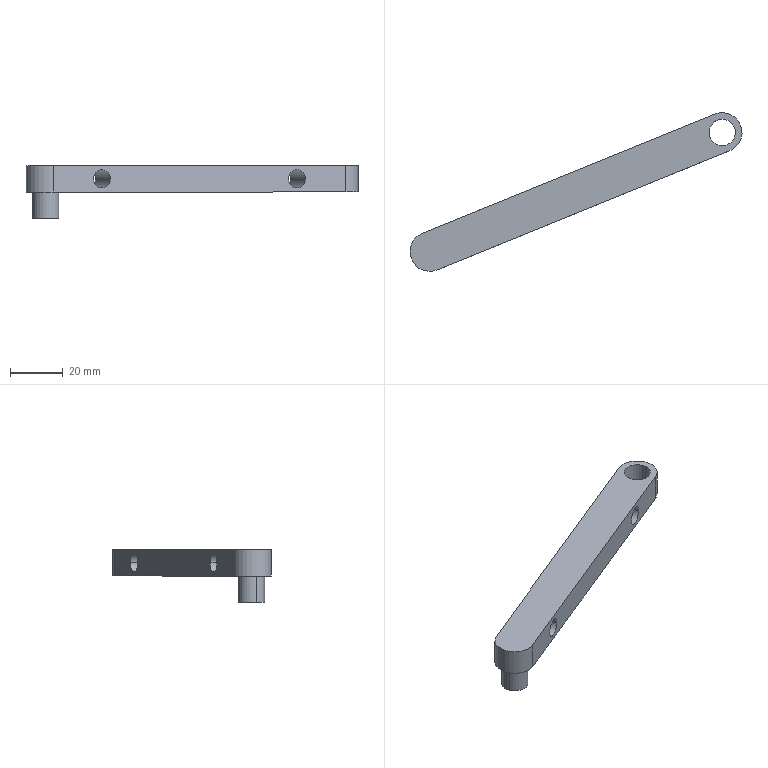Component | SolidWorks | ERocker(Left)-3 | 1 solid | 16 faces | box 126.14 x 60.24 x 20 mm | volume 18613 mm3 | cylinder 11 | plane 5 | commonest cylinder face diameters 7 x4 10 x4 15 x3
build123d program:
from build123d import *

# Parameters (mm, degrees)
BOSS_EXTRUDE1_DEPTH = 10
BOSS_EXTRUDE3_DEPTH = 10
SKETCH2_R           = 5
CUT_EXTRUDE1_DEPTH  = 10
SKETCH3_R           = 3.5
CUT_EXTRUDE2_DEPTH  = 16


with BuildPart() as part:
    # Sketch1_5 → Boss-Extrude1 (new body)
    with BuildSketch(Plane.XY):
        with BuildLine():
            Line((-95.746, 88.007), (-215.746, 88.007))
            ThreePointArc((-215.746, 88.007), (-223.246, 95.507), (-215.746, 103.007))
            Line((-215.746, 103.007), (-95.746, 103.007))
            ThreePointArc((-95.746, 103.007), (-88.246, 95.507), (-95.746, 88.007))
        make_face()
    extrude(amount=BOSS_EXTRUDE1_DEPTH)

    # Sketch1_5 2 → Boss-Extrude3 (add)
    with BuildSketch(Plane.XY):
        with BuildLine():
            ThreePointArc((-100.746, 95.507), (-95.746, 90.507), (-90.746, 95.507))
            ThreePointArc((-90.746, 95.507), (-95.746, 100.507), (-100.746, 95.507))
        make_face()
        with BuildLine():
            ThreePointArc((-100.746, 95.507), (-95.746, 90.507), (-90.746, 95.507))
            ThreePointArc((-90.746, 95.507), (-95.746, 100.507), (-100.746, 95.507))
        make_face()
    extrude(amount=-BOSS_EXTRUDE3_DEPTH)

    # Sketch2 → Cut-Extrude1 (cut)
    with BuildSketch(Plane.XY.offset(10)):
        with Locations((-215.746, 95.507)):
            Circle(SKETCH2_R)
    extrude(amount=-CUT_EXTRUDE1_DEPTH, mode=Mode.SUBTRACT)

    # Sketch3 → Cut-Extrude2 (cut)
    with BuildSketch(Plane(origin=(0, 103.007, 0), x_dir=(1, 0, 0), z_dir=(0, 1, 0))):
        with Locations(Location((-195.746, -5, 0), (0, 0, 180))):
            Circle(SKETCH3_R)
        with Locations(Location((-115.746, -5, 0), (0, 0, 180))):
            Circle(SKETCH3_R)
    extrude(amount=-CUT_EXTRUDE2_DEPTH, mode=Mode.SUBTRACT)


solid = part.part

# Placed as in the assembly
solid = solid.moved(Location((-64.373, 54.646, -27.818), (0, 0, -157.85)))
STEP:
#1=COLOUR_RGB('',0.7922,0.8196,0.9333);
#2=FILL_AREA_STYLE_COLOUR('',#1);
#3=FILL_AREA_STYLE('',(#2));
#4=SURFACE_STYLE_FILL_AREA(#3);
#5=SURFACE_SIDE_STYLE('',(#4));
#6=SURFACE_STYLE_USAGE(.BOTH.,#5);
#7=PRESENTATION_STYLE_ASSIGNMENT((#6));
#8=CARTESIAN_POINT('',(6.037,1.9,-0.8983));
#9=VERTEX_POINT('',#8);
#10=CARTESIAN_POINT('',(5.782,1.796,-0.8983));
#11=VERTEX_POINT('',#10);
#12=CARTESIAN_POINT('',(5.91,1.848,-0.8983));
#13=DIRECTION('',(-0.377,0.9262,0.));
#14=DIRECTION('',(-0.9262,-0.377,-0.));
#15=AXIS2_PLACEMENT_3D('',#12,#13,#14);
#16=CIRCLE('',#15,0.1378);
#17=EDGE_CURVE('',#9,#11,#16,.T.);
#18=ORIENTED_EDGE('',*,*,#17,.T.);
#19=CARTESIAN_POINT('',(6.005,1.249,-0.8983));
#20=VERTEX_POINT('',#19);
#21=CARTESIAN_POINT('',(5.767,1.832,-0.8983));
#22=DIRECTION('',(0.377,-0.9262,-0.));
#23=VECTOR('',#22,39.37);
#24=LINE('',#21,#23);
#25=EDGE_CURVE('',#11,#20,#24,.T.);
#26=ORIENTED_EDGE('',*,*,#25,.T.);
#27=CARTESIAN_POINT('',(6.26,1.353,-0.8983));
#28=VERTEX_POINT('',#27);
#29=CARTESIAN_POINT('',(6.132,1.301,-0.8983));
#30=DIRECTION('',(0.377,-0.9262,-0.));
#31=DIRECTION('',(0.9262,0.377,0.));
#32=AXIS2_PLACEMENT_3D('',#29,#30,#31);
#33=CIRCLE('',#32,0.1378);
#34=EDGE_CURVE('',#20,#28,#33,.T.);
#35=ORIENTED_EDGE('',*,*,#34,.T.);
#36=CARTESIAN_POINT('',(6.023,1.936,-0.8983));
#37=DIRECTION('',(0.377,-0.9262,-0.));
#38=VECTOR('',#37,39.37);
#39=LINE('',#36,#38);
#40=EDGE_CURVE('',#9,#28,#39,.T.);
#41=ORIENTED_EDGE('',*,*,#40,.F.);
#42=EDGE_LOOP('',(#18,#26,#35,#41));
#43=FACE_OUTER_BOUND('',#42,.T.);
#44=CARTESIAN_POINT('',(5.895,1.884,-0.8983));
#45=DIRECTION('',(0.377,-0.9262,-0.));
#46=DIRECTION('',(0.9262,0.377,0.));
#47=AXIS2_PLACEMENT_3D('',#44,#45,#46);
#48=CYLINDRICAL_SURFACE('',#47,0.1378);
#49=ADVANCED_FACE('',(#43),#48,.F.);
#50=CARTESIAN_POINT('',(3.12,0.7124,-0.8983));
#51=VERTEX_POINT('',#50);
#52=CARTESIAN_POINT('',(2.865,0.6084,-0.8983));
#53=VERTEX_POINT('',#52);
#54=CARTESIAN_POINT('',(2.993,0.6604,-0.8983));
#55=DIRECTION('',(-0.377,0.9262,0.));
#56=DIRECTION('',(-0.9262,-0.377,-0.));
#57=AXIS2_PLACEMENT_3D('',#54,#55,#56);
#58=CIRCLE('',#57,0.1378);
#59=EDGE_CURVE('',#51,#53,#58,.T.);
#60=ORIENTED_EDGE('',*,*,#59,.T.);
#61=CARTESIAN_POINT('',(3.088,0.06148,-0.8983));
#62=VERTEX_POINT('',#61);
#63=CARTESIAN_POINT('',(2.85,0.6449,-0.8983));
#64=DIRECTION('',(0.377,-0.9262,-0.));
#65=VECTOR('',#64,39.37);
#66=LINE('',#63,#65);
#67=EDGE_CURVE('',#53,#62,#66,.T.);
#68=ORIENTED_EDGE('',*,*,#67,.T.);
#69=CARTESIAN_POINT('',(3.343,0.1654,-0.8983));
#70=VERTEX_POINT('',#69);
#71=CARTESIAN_POINT('',(3.215,0.1134,-0.8983));
#72=DIRECTION('',(0.377,-0.9262,-0.));
#73=DIRECTION('',(0.9262,0.377,0.));
#74=AXIS2_PLACEMENT_3D('',#71,#72,#73);
#75=CIRCLE('',#74,0.1378);
#76=EDGE_CURVE('',#62,#70,#75,.T.);
#77=ORIENTED_EDGE('',*,*,#76,.T.);
#78=CARTESIAN_POINT('',(3.105,0.7488,-0.8983));
#79=DIRECTION('',(0.377,-0.9262,-0.));
#80=VECTOR('',#79,39.37);
#81=LINE('',#78,#80);
#82=EDGE_CURVE('',#51,#70,#81,.T.);
#83=ORIENTED_EDGE('',*,*,#82,.F.);
#84=EDGE_LOOP('',(#60,#68,#77,#83));
#85=FACE_OUTER_BOUND('',#84,.T.);
#86=CARTESIAN_POINT('',(2.978,0.6969,-0.8983));
#87=DIRECTION('',(0.377,-0.9262,-0.));
#88=DIRECTION('',(0.9262,0.377,0.));
#89=AXIS2_PLACEMENT_3D('',#86,#87,#88);
#90=CYLINDRICAL_SURFACE('',#89,0.1378);
#91=ADVANCED_FACE('',(#85),#90,.F.);
#92=CARTESIAN_POINT('',(6.933,1.946,-1.095));
#93=VERTEX_POINT('',#92);
#94=CARTESIAN_POINT('',(6.568,1.797,-1.095));
#95=VERTEX_POINT('',#94);
#96=CARTESIAN_POINT('',(6.75,1.871,-1.095));
#97=DIRECTION('',(-0.,-0.,1.));
#98=DIRECTION('',(-0.9262,-0.377,-0.));
#99=AXIS2_PLACEMENT_3D('',#96,#97,#98);
#100=CIRCLE('',#99,0.1969);
#101=EDGE_CURVE('',#93,#95,#100,.T.);
#102=ORIENTED_EDGE('',*,*,#101,.F.);
#103=CARTESIAN_POINT('',(6.933,1.946,-0.7015));
#104=VERTEX_POINT('',#103);
#105=CARTESIAN_POINT('',(6.933,1.946,-1.095));
#106=DIRECTION('',(-0.,-0.,1.));
#107=VECTOR('',#106,39.37);
#108=LINE('',#105,#107);
#109=EDGE_CURVE('',#93,#104,#108,.T.);
#110=ORIENTED_EDGE('',*,*,#109,.T.);
#111=CARTESIAN_POINT('',(6.568,1.797,-0.7015));
#112=VERTEX_POINT('',#111);
#113=CARTESIAN_POINT('',(6.75,1.871,-0.7015));
#114=DIRECTION('',(-0.,-0.,1.));
#115=DIRECTION('',(-0.9262,-0.377,-0.));
#116=AXIS2_PLACEMENT_3D('',#113,#114,#115);
#117=CIRCLE('',#116,0.1969);
#118=EDGE_CURVE('',#104,#112,#117,.T.);
#119=ORIENTED_EDGE('',*,*,#118,.T.);
#120=CARTESIAN_POINT('',(6.568,1.797,-1.095));
#121=DIRECTION('',(-0.,-0.,1.));
#122=VECTOR('',#121,39.37);
#123=LINE('',#120,#122);
#124=EDGE_CURVE('',#95,#112,#123,.T.);
#125=ORIENTED_EDGE('',*,*,#124,.F.);
#126=EDGE_LOOP('',(#102,#110,#119,#125));
#127=FACE_OUTER_BOUND('',#126,.T.);
#128=CARTESIAN_POINT('',(6.75,1.871,-1.095));
#129=DIRECTION('',(-0.,-0.,1.));
#130=DIRECTION('',(-0.9262,-0.377,-0.));
#131=AXIS2_PLACEMENT_3D('',#128,#129,#130);
#132=CYLINDRICAL_SURFACE('',#131,0.1969);
#133=ADVANCED_FACE('',(#127),#132,.F.);
#134=CARTESIAN_POINT('',(2.192,0.01582,-1.489));
#135=VERTEX_POINT('',#134);
#136=CARTESIAN_POINT('',(2.557,0.1643,-1.489));
#137=VERTEX_POINT('',#136);
#138=CARTESIAN_POINT('',(2.375,0.09004,-1.489));
#139=DIRECTION('',(-0.,-0.,1.));
#140=DIRECTION('',(-0.9262,-0.377,0.));
#141=AXIS2_PLACEMENT_3D('',#138,#139,#140);
#142=CIRCLE('',#141,0.1969);
#143=EDGE_CURVE('',#135,#137,#142,.T.);
#144=ORIENTED_EDGE('',*,*,#143,.T.);
#145=CARTESIAN_POINT('',(2.557,0.1643,-1.095));
#146=VERTEX_POINT('',#145);
#147=CARTESIAN_POINT('',(2.557,0.1643,-1.489));
#148=DIRECTION('',(-0.,-0.,1.));
#149=VECTOR('',#148,39.37);
#150=LINE('',#147,#149);
#151=EDGE_CURVE('',#137,#146,#150,.T.);
#152=ORIENTED_EDGE('',*,*,#151,.T.);
#153=CARTESIAN_POINT('',(2.192,0.01582,-1.095));
#154=VERTEX_POINT('',#153);
#155=CARTESIAN_POINT('',(2.375,0.09004,-1.095));
#156=DIRECTION('',(-0.,-0.,1.));
#157=DIRECTION('',(-0.9262,-0.377,-0.));
#158=AXIS2_PLACEMENT_3D('',#155,#156,#157);
#159=CIRCLE('',#158,0.1969);
#160=EDGE_CURVE('',#154,#146,#159,.T.);
#161=ORIENTED_EDGE('',*,*,#160,.F.);
#162=CARTESIAN_POINT('',(2.192,0.01582,-1.489));
#163=DIRECTION('',(-0.,-0.,1.));
#164=VECTOR('',#163,39.37);
#165=LINE('',#162,#164);
#166=EDGE_CURVE('',#135,#154,#165,.T.);
#167=ORIENTED_EDGE('',*,*,#166,.F.);
#168=EDGE_LOOP('',(#144,#152,#161,#167));
#169=FACE_OUTER_BOUND('',#168,.T.);
#170=CARTESIAN_POINT('',(2.375,0.09004,-1.489));
#171=DIRECTION('',(-0.,-0.,1.));
#172=DIRECTION('',(-0.9262,-0.377,0.));
#173=AXIS2_PLACEMENT_3D('',#170,#171,#172);
#174=CYLINDRICAL_SURFACE('',#173,0.1969);
#175=ADVANCED_FACE('',(#169),#174,.T.);
#176=CARTESIAN_POINT('',(7.024,1.983,-0.7015));
#177=VERTEX_POINT('',#176);
#178=CARTESIAN_POINT('',(6.639,2.145,-0.7015));
#179=VERTEX_POINT('',#178);
#180=CARTESIAN_POINT('',(6.75,1.871,-0.7015));
#181=DIRECTION('',(-0.,-0.,1.));
#182=DIRECTION('',(-0.9262,-0.377,-0.));
#183=AXIS2_PLACEMENT_3D('',#180,#181,#182);
#184=CIRCLE('',#183,0.2953);
#185=EDGE_CURVE('',#177,#179,#184,.T.);
#186=ORIENTED_EDGE('',*,*,#185,.F.);
#187=CARTESIAN_POINT('',(7.024,1.983,-1.095));
#188=VERTEX_POINT('',#187);
#189=CARTESIAN_POINT('',(7.024,1.983,-0.7015));
#190=DIRECTION('',(0.,0.,-1.));
#191=VECTOR('',#190,39.37);
#192=LINE('',#189,#191);
#193=EDGE_CURVE('',#177,#188,#192,.T.);
#194=ORIENTED_EDGE('',*,*,#193,.T.);
#195=CARTESIAN_POINT('',(6.639,2.145,-1.095));
#196=VERTEX_POINT('',#195);
#197=CARTESIAN_POINT('',(6.75,1.871,-1.095));
#198=DIRECTION('',(-0.,-0.,1.));
#199=DIRECTION('',(-0.9262,-0.377,-0.));
#200=AXIS2_PLACEMENT_3D('',#197,#198,#199);
#201=CIRCLE('',#200,0.2953);
#202=EDGE_CURVE('',#188,#196,#201,.T.);
#203=ORIENTED_EDGE('',*,*,#202,.T.);
#204=CARTESIAN_POINT('',(6.639,2.145,-0.7015));
#205=DIRECTION('',(0.,0.,-1.));
#206=VECTOR('',#205,39.37);
#207=LINE('',#204,#206);
#208=EDGE_CURVE('',#179,#196,#207,.T.);
#209=ORIENTED_EDGE('',*,*,#208,.F.);
#210=EDGE_LOOP('',(#186,#194,#203,#209));
#211=FACE_OUTER_BOUND('',#210,.T.);
#212=CARTESIAN_POINT('',(6.75,1.871,-0.7015));
#213=DIRECTION('',(0.,0.,-1.));
#214=DIRECTION('',(0.9262,0.377,0.));
#215=AXIS2_PLACEMENT_3D('',#212,#213,#214);
#216=CYLINDRICAL_SURFACE('',#215,0.2953);
#217=ADVANCED_FACE('',(#211),#216,.T.);
#218=CARTESIAN_POINT('',(6.75,1.871,-0.7015));
#219=DIRECTION('',(-0.,-0.,1.));
#220=DIRECTION('',(-0.9262,-0.377,-0.));
#221=AXIS2_PLACEMENT_3D('',#218,#219,#220);
#222=CIRCLE('',#221,0.1969);
#223=EDGE_CURVE('',#112,#104,#222,.T.);
#224=ORIENTED_EDGE('',*,*,#223,.F.);
#225=ORIENTED_EDGE('',*,*,#118,.F.);
#226=EDGE_LOOP('',(#224,#225));
#227=FACE_BOUND('',#226,.T.);
#228=CARTESIAN_POINT('',(2.486,-0.1834,-0.7015));
#229=VERTEX_POINT('',#228);
#230=CARTESIAN_POINT('',(6.862,1.598,-0.7015));
#231=VERTEX_POINT('',#230);
#232=CARTESIAN_POINT('',(-1.005,-1.605,-0.7015));
#233=DIRECTION('',(0.9262,0.377,0.));
#234=VECTOR('',#233,39.37);
#235=LINE('',#232,#234);
#236=EDGE_CURVE('',#229,#231,#235,.T.);
#237=ORIENTED_EDGE('',*,*,#236,.T.);
#238=CARTESIAN_POINT('',(6.75,1.871,-0.7015));
#239=DIRECTION('',(-0.,-0.,1.));
#240=DIRECTION('',(-0.9262,-0.377,-0.));
#241=AXIS2_PLACEMENT_3D('',#238,#239,#240);
#242=CIRCLE('',#241,0.2953);
#243=EDGE_CURVE('',#231,#177,#242,.T.);
#244=ORIENTED_EDGE('',*,*,#243,.T.);
#245=ORIENTED_EDGE('',*,*,#185,.T.);
#246=CARTESIAN_POINT('',(2.263,0.3635,-0.7015));
#247=VERTEX_POINT('',#246);
#248=CARTESIAN_POINT('',(-1.228,-1.058,-0.7015));
#249=DIRECTION('',(0.9262,0.377,0.));
#250=VECTOR('',#249,39.37);
#251=LINE('',#248,#250);
#252=EDGE_CURVE('',#247,#179,#251,.T.);
#253=ORIENTED_EDGE('',*,*,#252,.F.);
#254=CARTESIAN_POINT('',(2.375,0.09004,-0.7015));
#255=DIRECTION('',(-0.,-0.,1.));
#256=DIRECTION('',(-0.9262,-0.377,-0.));
#257=AXIS2_PLACEMENT_3D('',#254,#255,#256);
#258=CIRCLE('',#257,0.2953);
#259=EDGE_CURVE('',#247,#229,#258,.T.);
#260=ORIENTED_EDGE('',*,*,#259,.T.);
#261=EDGE_LOOP('',(#237,#244,#245,#253,#260));
#262=FACE_OUTER_BOUND('',#261,.T.);
#263=CARTESIAN_POINT('',(-2.534,2.151,-0.7015));
#264=DIRECTION('',(-0.,-0.,1.));
#265=DIRECTION('',(-0.9262,-0.377,-0.));
#266=AXIS2_PLACEMENT_3D('',#263,#264,#265);
#267=PLANE('',#266);
#268=ADVANCED_FACE('',(#227,#262),#267,.T.);
#269=CARTESIAN_POINT('',(6.75,1.871,-1.095));
#270=DIRECTION('',(-0.,-0.,1.));
#271=DIRECTION('',(-0.9262,-0.377,-0.));
#272=AXIS2_PLACEMENT_3D('',#269,#270,#271);
#273=CIRCLE('',#272,0.1969);
#274=EDGE_CURVE('',#95,#93,#273,.T.);
#275=ORIENTED_EDGE('',*,*,#274,.T.);
#276=ORIENTED_EDGE('',*,*,#101,.T.);
#277=EDGE_LOOP('',(#275,#276));
#278=FACE_BOUND('',#277,.T.);
#279=ORIENTED_EDGE('',*,*,#160,.T.);
#280=CARTESIAN_POINT('',(2.375,0.09004,-1.095));
#281=DIRECTION('',(-0.,-0.,1.));
#282=DIRECTION('',(-0.9262,-0.377,-0.));
#283=AXIS2_PLACEMENT_3D('',#280,#281,#282);
#284=CIRCLE('',#283,0.1969);
#285=EDGE_CURVE('',#146,#154,#284,.T.);
#286=ORIENTED_EDGE('',*,*,#285,.T.);
#287=EDGE_LOOP('',(#279,#286));
#288=FACE_BOUND('',#287,.T.);
#289=CARTESIAN_POINT('',(2.486,-0.1834,-1.095));
#290=VERTEX_POINT('',#289);
#291=CARTESIAN_POINT('',(6.862,1.598,-1.095));
#292=VERTEX_POINT('',#291);
#293=CARTESIAN_POINT('',(-1.005,-1.605,-1.095));
#294=DIRECTION('',(0.9262,0.377,0.));
#295=VECTOR('',#294,39.37);
#296=LINE('',#293,#295);
#297=EDGE_CURVE('',#290,#292,#296,.T.);
#298=ORIENTED_EDGE('',*,*,#297,.F.);
#299=CARTESIAN_POINT('',(2.263,0.3635,-1.095));
#300=VERTEX_POINT('',#299);
#301=CARTESIAN_POINT('',(2.375,0.09004,-1.095));
#302=DIRECTION('',(-0.,-0.,1.));
#303=DIRECTION('',(-0.9262,-0.377,-0.));
#304=AXIS2_PLACEMENT_3D('',#301,#302,#303);
#305=CIRCLE('',#304,0.2953);
#306=EDGE_CURVE('',#300,#290,#305,.T.);
#307=ORIENTED_EDGE('',*,*,#306,.F.);
#308=CARTESIAN_POINT('',(-1.228,-1.058,-1.095));
#309=DIRECTION('',(0.9262,0.377,0.));
#310=VECTOR('',#309,39.37);
#311=LINE('',#308,#310);
#312=EDGE_CURVE('',#300,#196,#311,.T.);
#313=ORIENTED_EDGE('',*,*,#312,.T.);
#314=ORIENTED_EDGE('',*,*,#202,.F.);
#315=CARTESIAN_POINT('',(6.75,1.871,-1.095));
#316=DIRECTION('',(-0.,-0.,1.));
#317=DIRECTION('',(-0.9262,-0.377,-0.));
#318=AXIS2_PLACEMENT_3D('',#315,#316,#317);
#319=CIRCLE('',#318,0.2953);
#320=EDGE_CURVE('',#292,#188,#319,.T.);
#321=ORIENTED_EDGE('',*,*,#320,.F.);
#322=EDGE_LOOP('',(#298,#307,#313,#314,#321));
#323=FACE_OUTER_BOUND('',#322,.T.);
#324=CARTESIAN_POINT('',(-2.534,2.151,-1.095));
#325=DIRECTION('',(-0.,-0.,1.));
#326=DIRECTION('',(-0.9262,-0.377,-0.));
#327=AXIS2_PLACEMENT_3D('',#324,#325,#326);
#328=PLANE('',#327);
#329=ADVANCED_FACE('',(#278,#288,#323),#328,.F.);
#330=ORIENTED_EDGE('',*,*,#193,.F.);
#331=ORIENTED_EDGE('',*,*,#243,.F.);
#332=CARTESIAN_POINT('',(6.862,1.598,-0.7015));
#333=DIRECTION('',(0.,0.,-1.));
#334=VECTOR('',#333,39.37);
#335=LINE('',#332,#334);
#336=EDGE_CURVE('',#231,#292,#335,.T.);
#337=ORIENTED_EDGE('',*,*,#336,.T.);
#338=ORIENTED_EDGE('',*,*,#320,.T.);
#339=EDGE_LOOP('',(#330,#331,#337,#338));
#340=FACE_OUTER_BOUND('',#339,.T.);
#341=CARTESIAN_POINT('',(6.75,1.871,-0.7015));
#342=DIRECTION('',(0.,0.,-1.));
#343=DIRECTION('',(0.9262,0.377,0.));
#344=AXIS2_PLACEMENT_3D('',#341,#342,#343);
#345=CYLINDRICAL_SURFACE('',#344,0.2953);
#346=ADVANCED_FACE('',(#340),#345,.T.);
#347=ORIENTED_EDGE('',*,*,#17,.F.);
#348=CARTESIAN_POINT('',(5.91,1.848,-0.8983));
#349=DIRECTION('',(-0.377,0.9262,0.));
#350=DIRECTION('',(-0.9262,-0.377,-0.));
#351=AXIS2_PLACEMENT_3D('',#348,#349,#350);
#352=CIRCLE('',#351,0.1378);
#353=EDGE_CURVE('',#11,#9,#352,.T.);
#354=ORIENTED_EDGE('',*,*,#353,.F.);
#355=EDGE_LOOP('',(#347,#354));
#356=FACE_BOUND('',#355,.T.);
#357=ORIENTED_EDGE('',*,*,#59,.F.);
#358=CARTESIAN_POINT('',(2.993,0.6604,-0.8983));
#359=DIRECTION('',(-0.377,0.9262,0.));
#360=DIRECTION('',(-0.9262,-0.377,-0.));
#361=AXIS2_PLACEMENT_3D('',#358,#359,#360);
#362=CIRCLE('',#361,0.1378);
#363=EDGE_CURVE('',#53,#51,#362,.T.);
#364=ORIENTED_EDGE('',*,*,#363,.F.);
#365=EDGE_LOOP('',(#357,#364));
#366=FACE_BOUND('',#365,.T.);
#367=ORIENTED_EDGE('',*,*,#312,.F.);
#368=CARTESIAN_POINT('',(2.263,0.3635,-0.7015));
#369=DIRECTION('',(0.,0.,-1.));
#370=VECTOR('',#369,39.37);
#371=LINE('',#368,#370);
#372=EDGE_CURVE('',#247,#300,#371,.T.);
#373=ORIENTED_EDGE('',*,*,#372,.F.);
#374=ORIENTED_EDGE('',*,*,#252,.T.);
#375=ORIENTED_EDGE('',*,*,#208,.T.);
#376=EDGE_LOOP('',(#367,#373,#374,#375));
#377=FACE_OUTER_BOUND('',#376,.T.);
#378=CARTESIAN_POINT('',(-1.228,-1.058,-0.7015));
#379=DIRECTION('',(-0.377,0.9262,0.));
#380=DIRECTION('',(-0.9262,-0.377,-0.));
#381=AXIS2_PLACEMENT_3D('',#378,#379,#380);
#382=PLANE('',#381);
#383=ADVANCED_FACE('',(#356,#366,#377),#382,.T.);
#384=ORIENTED_EDGE('',*,*,#306,.T.);
#385=CARTESIAN_POINT('',(2.486,-0.1834,-0.7015));
#386=DIRECTION('',(0.,0.,-1.));
#387=VECTOR('',#386,39.37);
#388=LINE('',#385,#387);
#389=EDGE_CURVE('',#229,#290,#388,.T.);
#390=ORIENTED_EDGE('',*,*,#389,.F.);
#391=ORIENTED_EDGE('',*,*,#259,.F.);
#392=ORIENTED_EDGE('',*,*,#372,.T.);
#393=EDGE_LOOP('',(#384,#390,#391,#392));
#394=FACE_OUTER_BOUND('',#393,.T.);
#395=CARTESIAN_POINT('',(2.375,0.09004,-0.7015));
#396=DIRECTION('',(0.,0.,-1.));
#397=DIRECTION('',(0.9262,0.377,0.));
#398=AXIS2_PLACEMENT_3D('',#395,#396,#397);
#399=CYLINDRICAL_SURFACE('',#398,0.2953);
#400=ADVANCED_FACE('',(#394),#399,.T.);
#401=CARTESIAN_POINT('',(6.132,1.301,-0.8983));
#402=DIRECTION('',(0.377,-0.9262,-0.));
#403=DIRECTION('',(0.9262,0.377,0.));
#404=AXIS2_PLACEMENT_3D('',#401,#402,#403);
#405=CIRCLE('',#404,0.1378);
#406=EDGE_CURVE('',#28,#20,#405,.T.);
#407=ORIENTED_EDGE('',*,*,#406,.F.);
#408=ORIENTED_EDGE('',*,*,#34,.F.);
#409=EDGE_LOOP('',(#407,#408));
#410=FACE_BOUND('',#409,.T.);
#411=CARTESIAN_POINT('',(3.215,0.1134,-0.8983));
#412=DIRECTION('',(0.377,-0.9262,-0.));
#413=DIRECTION('',(0.9262,0.377,0.));
#414=AXIS2_PLACEMENT_3D('',#411,#412,#413);
#415=CIRCLE('',#414,0.1378);
#416=EDGE_CURVE('',#70,#62,#415,.T.);
#417=ORIENTED_EDGE('',*,*,#416,.F.);
#418=ORIENTED_EDGE('',*,*,#76,.F.);
#419=EDGE_LOOP('',(#417,#418));
#420=FACE_BOUND('',#419,.T.);
#421=ORIENTED_EDGE('',*,*,#297,.T.);
#422=ORIENTED_EDGE('',*,*,#336,.F.);
#423=ORIENTED_EDGE('',*,*,#236,.F.);
#424=ORIENTED_EDGE('',*,*,#389,.T.);
#425=EDGE_LOOP('',(#421,#422,#423,#424));
#426=FACE_OUTER_BOUND('',#425,.T.);
#427=CARTESIAN_POINT('',(-1.005,-1.605,-0.7015));
#428=DIRECTION('',(-0.377,0.9262,0.));
#429=DIRECTION('',(-0.9262,-0.377,-0.));
#430=AXIS2_PLACEMENT_3D('',#427,#428,#429);
#431=PLANE('',#430);
#432=ADVANCED_FACE('',(#410,#420,#426),#431,.F.);
#433=ORIENTED_EDGE('',*,*,#151,.F.);
#434=CARTESIAN_POINT('',(2.375,0.09004,-1.489));
#435=DIRECTION('',(-0.,-0.,1.));
#436=DIRECTION('',(-0.9262,-0.377,0.));
#437=AXIS2_PLACEMENT_3D('',#434,#435,#436);
#438=CIRCLE('',#437,0.1969);
#439=EDGE_CURVE('',#137,#135,#438,.T.);
#440=ORIENTED_EDGE('',*,*,#439,.T.);
#441=ORIENTED_EDGE('',*,*,#166,.T.);
#442=ORIENTED_EDGE('',*,*,#285,.F.);
#443=EDGE_LOOP('',(#433,#440,#441,#442));
#444=FACE_OUTER_BOUND('',#443,.T.);
#445=CARTESIAN_POINT('',(2.375,0.09004,-1.489));
#446=DIRECTION('',(-0.,-0.,1.));
#447=DIRECTION('',(-0.9262,-0.377,0.));
#448=AXIS2_PLACEMENT_3D('',#445,#446,#447);
#449=CYLINDRICAL_SURFACE('',#448,0.1969);
#450=ADVANCED_FACE('',(#444),#449,.T.);
#451=ORIENTED_EDGE('',*,*,#143,.F.);
#452=ORIENTED_EDGE('',*,*,#439,.F.);
#453=EDGE_LOOP('',(#451,#452));
#454=FACE_OUTER_BOUND('',#453,.T.);
#455=CARTESIAN_POINT('',(-2.534,2.151,-1.489));
#456=DIRECTION('',(-0.,-0.,1.));
#457=DIRECTION('',(-0.9262,-0.377,-0.));
#458=AXIS2_PLACEMENT_3D('',#455,#456,#457);
#459=PLANE('',#458);
#460=ADVANCED_FACE('',(#454),#459,.F.);
#461=ORIENTED_EDGE('',*,*,#109,.F.);
#462=ORIENTED_EDGE('',*,*,#274,.F.);
#463=ORIENTED_EDGE('',*,*,#124,.T.);
#464=ORIENTED_EDGE('',*,*,#223,.T.);
#465=EDGE_LOOP('',(#461,#462,#463,#464));
#466=FACE_OUTER_BOUND('',#465,.T.);
#467=CARTESIAN_POINT('',(6.75,1.871,-1.095));
#468=DIRECTION('',(-0.,-0.,1.));
#469=DIRECTION('',(-0.9262,-0.377,-0.));
#470=AXIS2_PLACEMENT_3D('',#467,#468,#469);
#471=CYLINDRICAL_SURFACE('',#470,0.1969);
#472=ADVANCED_FACE('',(#466),#471,.F.);
#473=ORIENTED_EDGE('',*,*,#67,.F.);
#474=ORIENTED_EDGE('',*,*,#363,.T.);
#475=ORIENTED_EDGE('',*,*,#82,.T.);
#476=ORIENTED_EDGE('',*,*,#416,.T.);
#477=EDGE_LOOP('',(#473,#474,#475,#476));
#478=FACE_OUTER_BOUND('',#477,.T.);
#479=CARTESIAN_POINT('',(2.978,0.6969,-0.8983));
#480=DIRECTION('',(0.377,-0.9262,-0.));
#481=DIRECTION('',(0.9262,0.377,0.));
#482=AXIS2_PLACEMENT_3D('',#479,#480,#481);
#483=CYLINDRICAL_SURFACE('',#482,0.1378);
#484=ADVANCED_FACE('',(#478),#483,.F.);
#485=ORIENTED_EDGE('',*,*,#25,.F.);
#486=ORIENTED_EDGE('',*,*,#353,.T.);
#487=ORIENTED_EDGE('',*,*,#40,.T.);
#488=ORIENTED_EDGE('',*,*,#406,.T.);
#489=EDGE_LOOP('',(#485,#486,#487,#488));
#490=FACE_OUTER_BOUND('',#489,.T.);
#491=CARTESIAN_POINT('',(5.895,1.884,-0.8983));
#492=DIRECTION('',(0.377,-0.9262,-0.));
#493=DIRECTION('',(0.9262,0.377,0.));
#494=AXIS2_PLACEMENT_3D('',#491,#492,#493);
#495=CYLINDRICAL_SURFACE('',#494,0.1378);
#496=ADVANCED_FACE('',(#490),#495,.F.);
#497=CLOSED_SHELL('',(#49,#91,#133,#175,#217,#268,#329,#346,#383,#400,#432,#450,#460,#472,#484,#496));
#498=MANIFOLD_SOLID_BREP('',#497);
#499=STYLED_ITEM('',(#7),#498);
#500=PRESENTATION_LAYER_ASSIGNMENT('','',(#499));
#501=(LENGTH_UNIT()NAMED_UNIT(*)SI_UNIT($,.METRE.));
#502=LENGTH_MEASURE_WITH_UNIT(LENGTH_MEASURE(0.0254),#501);
#503=DIMENSIONAL_EXPONENTS(1.,0.,0.,0.,0.,0.,0.);
#504=(CONVERSION_BASED_UNIT('',#502)LENGTH_UNIT()NAMED_UNIT(#503));
#505=UNCERTAINTY_MEASURE_WITH_UNIT(LENGTH_MEASURE(0.00001),#504,'','');
#506=(NAMED_UNIT(*)PLANE_ANGLE_UNIT()SI_UNIT($,.RADIAN.));
#507=(NAMED_UNIT(*)SI_UNIT($,.STERADIAN.)SOLID_ANGLE_UNIT());
#508=(GEOMETRIC_REPRESENTATION_CONTEXT(3)GLOBAL_UNCERTAINTY_ASSIGNED_CONTEXT((#505))GLOBAL_UNIT_ASSIGNED_CONTEXT((#504,#506,#507))REPRESENTATION_CONTEXT('',''));
#509=MECHANICAL_DESIGN_GEOMETRIC_PRESENTATION_REPRESENTATION('',(#499),#508);
#510=CARTESIAN_POINT('',(0.,0.,0.));
#511=DIRECTION('',(0.,0.,1.));
#512=DIRECTION('',(1.,0.,0.));
#513=AXIS2_PLACEMENT_3D('',#510,#511,#512);
#514=(LENGTH_UNIT()NAMED_UNIT(*)SI_UNIT($,.METRE.));
#515=LENGTH_MEASURE_WITH_UNIT(LENGTH_MEASURE(0.0254),#514);
#516=DIMENSIONAL_EXPONENTS(1.,0.,0.,0.,0.,0.,0.);
#517=(CONVERSION_BASED_UNIT('',#515)LENGTH_UNIT()NAMED_UNIT(#516));
#518=UNCERTAINTY_MEASURE_WITH_UNIT(LENGTH_MEASURE(0.00001),#517,'','');
#519=(NAMED_UNIT(*)PLANE_ANGLE_UNIT()SI_UNIT($,.RADIAN.));
#520=(NAMED_UNIT(*)SI_UNIT($,.STERADIAN.)SOLID_ANGLE_UNIT());
#521=(GEOMETRIC_REPRESENTATION_CONTEXT(3)GLOBAL_UNCERTAINTY_ASSIGNED_CONTEXT((#518))GLOBAL_UNIT_ASSIGNED_CONTEXT((#517,#519,#520))REPRESENTATION_CONTEXT('',''));
#522=ADVANCED_BREP_SHAPE_REPRESENTATION('',(#498,#513),#521);